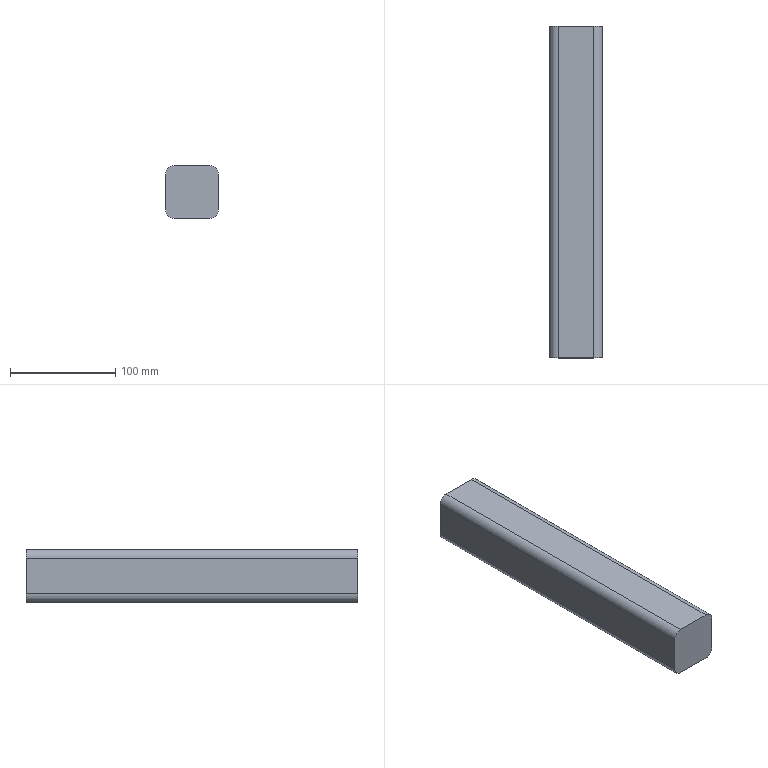Component | SolidWorks | AX00-100.1.1-1_AXFrame_A.1.1-1_AX50x50-6_square tube.1.1-1 | 1 solid | 20 faces | box 50 x 315 x 50 mm | volume 284551 mm3 | plane 12 | cylinder 8 | commonest cylinder face diameters 16 x4 6 x4 | material AISI 1035 Steel (SS)
build123d program:
from build123d import *

# Parameters (mm, degrees)
SKETCH1_W           = 50
SKETCH1_H           = 50
BOSS_EXTRUDE1_DEPTH = 157.5
FILLET3_R           = 8
SHELL1_T            = 5


with BuildPart() as part:
    # Sketch1 → Boss-Extrude1 (new, symmetric)
    with BuildSketch(Plane.XY):
        Rectangle(SKETCH1_W, SKETCH1_H)
    extrude(amount=BOSS_EXTRUDE1_DEPTH, both=True)

    # Fillet3
    fillet3_edges = [part.edges().sort_by_distance(p)[0] for p in [
        (25, -25, 0),
        (-25, -25, 0),
        (-25, 25, 0),
        (25, 25, 0),
    ]]
    fillet(fillet3_edges, radius=FILLET3_R)

    # Shell1 (no face opened: a closed hollow body)
    add(offset(amount=-SHELL1_T, mode=Mode.PRIVATE), mode=Mode.SUBTRACT)


solid = part.part

# Placed as in the assembly
solid = solid.moved(Location((-116.369, 1305.864, 187.5), (90, 0, 0)))